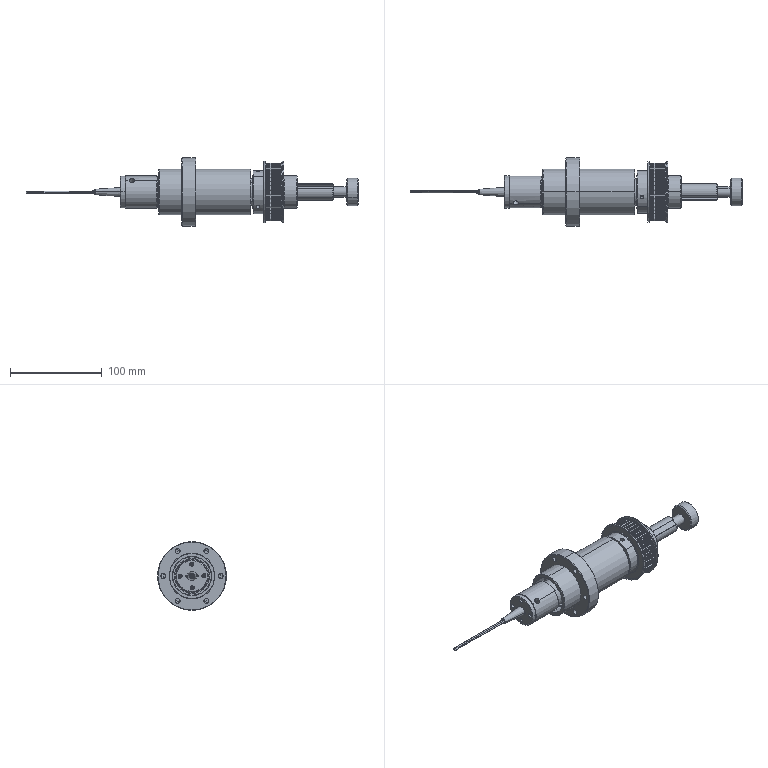Assembly | SolidWorks | mm | 15 component files | 15 solids | 1172 faces | box 362 x 75 x 75 mm | volume 344759 mm3 | cylinder 608 | torus 202 | cone 131 | plane 125 | sphere 104 | spline 2 | commonest cylinder face diameters 1.1 x98 0.5 x92 6.55 x86 59.16 x41 62.7 x40 5.5 x20 6 x20 3.4 x18
Bill of materials:
deep groove ball bearings gb | 4 |  | Ring-and-ball assembly geometry: an outer ring and an inner ring, concentric, with a row of spherical balls between them. The overall shape looks like a rolling-element ball bearing.
FlatKey6-175 | 1 | Alternative Material | Long, slender bar with a rectangular cross-section and five evenly spaced small round holes in a line along its length.
HTPA40S5M150_B_H30 | 1 | 45# | Toothed pulley-like rotational part: a cylindrical body with straight axial teeth around its outside, a thin flange at each end of the toothed section, and a smaller cylindrical hub on one side. It has a through bore with one keyway, and radial holes go through the hub wall.
JJDJR-3060-E-001 | 1 | 45# | Hollow cylindrical sleeve with a single circular flange placed off-center along its length. The flange has six through holes on a bolt circle.
JJDJR-3060-E-002 | 1 | 40Cr | Long hollow tube with a larger-diameter collar at one end, a row of small radial holes along its length, a slot near the other end, and a keyed bore.
JJDJR-3060-E-003 | 1 | 45# | Thick annular ring with chamfered outer edges, a central bore, and eight axial through holes evenly spaced around it.
JJDJR-3060-E-004 | 1 | 40Cr | Long shaft with a flat along its body, a smaller-diameter pin at one end with an axial hole, and a notched end block with small cross holes at the other end.
JJDJR-3060-E-005 | 1 | Tungsten Alloy | Thick plain washer- or spacer-like ring with chamfered outer edges and a small central through hole.
JJDJR-3060-E-006 | 1 | 40Cr | Small block with one convex curved face and a stepped rectangular tongue on the opposite side, pierced by two counterbored holes.
JJDJR-3060-E-007 | 1 | 40Cr | Circular flange with a long tapered conical shank on one side and a short stepped pilot boss on the other side.
JJDJR-3060-E-025 | 1 | Aluminum Alloy | Long thin rod with a slightly larger cylindrical hub at one end. The hub has a flat or notch, and the opposite end has a chamfered, slightly tapered tip.
Key6X6-36 | 1 | Alternative Material | Small rectangular bar with fully rounded ends (obround outline) and small chamfers along the edges.
Mates:
1. coincident | JJDJR-3060-E-001-1 face at (-89.59, -8.263, -16.52) dir (-1, 0, 0) | deep groove ball bearings gb-1 face at (-89.59, -41.121, -21.847) dir (1, 0, 0)
2. concentric | JJDJR-3060-E-001-1 face at (-103.59, -29.263, -16.52) dir (-1, 0, 0) r 21 | deep groove ball bearings gb-1 face at (-102.301, -29.263, -16.52) dir (-1, 0, 0) r 13
3. concentric | JJDJR-3060-E-001-1 face at (-103.59, -29.263, -16.52) dir (-1, 0, 0) r 21 | deep groove ball bearings gb-2 face at (-110.301, -29.263, -16.52) dir (-1, 0, 0) r 13
4. coincident | JJDJR-3060-E-001-1 face at (-17.59, -8.263, -16.52) dir (1, 0, 0) | deep groove ball bearings gb-3 face at (-17.59, -16.263, -16.52) dir (-1, 0, 0)
5. concentric | JJDJR-3060-E-001-1 face at (-103.59, -29.263, -16.52) dir (-1, 0, 0) r 21 | deep groove ball bearings gb-3 face at (-22.301, -29.263, -16.52) dir (-1, 0, 0) r 13
6. coincident | JJDJR-3060-E-002-1 face at (22.41, -37.957, -24.791) dir (0, -0.7245, -0.6892) | Key6X6-36-1 face at (22.41, -37.957, -24.791) dir (0, 0.7245, 0.6892)
7. concentric | JJDJR-3060-E-002-1 face at (34.41, -29.562, -28.516) dir (1, 0, 0) r 1.25 | JJDJR-3060-E-003-1 face at (47.41, -29.562, -28.516) dir (1, 0, 0) r 1.7
8. concentric | JJDJR-3060-E-002-1 face at (-140.59, -28.938, -3.524) dir (-1, 0, 0) r 1.65 | JJDJR-3060-E-007-1 face at (-137.59, -28.938, -3.524) dir (-1, 0, 0) r 2.25
9. concentric | JJDJR-3060-E-002-1 face at (22.41, -45.202, -31.684) dir (0, 0.7245, 0.6892) r 3 | Key6X6-36-1 face at (22.41, -42.304, -28.927) dir (0, 0.7245, 0.6892) r 3
10. concentric | JJDJR-3060-E-002-1 face at (-1.59, -45.202, -31.684) dir (0, 0.7245, 0.6892) r 3 | Key6X6-36-1 face at (-1.59, -42.304, -28.927) dir (0, 0.7245, 0.6892) r 3
11. concentric | JJDJR-3060-E-002-1 face at (-140.59, -29.263, -16.52) dir (-1, 0, 0) r 15 | deep groove ball bearings gb-2 face at (-108.562, -29.263, -16.52) dir (-1, 0, 0) r 5
12. concentric | JJDJR-3060-E-002-1 face at (-140.59, -29.263, -16.52) dir (-1, 0, 0) r 15 | HTPA40S5M150_B_H30-2 face at (-1.59, -29.263, -16.52) dir (1, 0, 0) r 15
13. coincident | JJDJR-3060-E-002-1 face at (-140.59, -33.61, -20.656) dir (-1, 0, 0) | JJDJR-3060-E-007-1 face at (-140.59, -29.038, -7.523) dir (1, 0, 0)
14. concentric | JJDJR-3060-E-002-1 face at (-140.59, -29.587, -29.516) dir (-1, 0, 0) r 1.65 | JJDJR-3060-E-007-1 face at (-137.59, -29.587, -29.516) dir (-1, 0, 0) r 2.25
15. coincident | JJDJR-3060-E-002-1 face at (-105.59, -41.942, -28.582) dir (1, 0, 0) | deep groove ball bearings gb-2 face at (-105.59, -36.929, -16.52) dir (-1, 0, 0)
16. concentric | JJDJR-3060-E-002-1 face at (34.41, -28.963, -4.524) dir (1, 0, 0) r 1.25 | JJDJR-3060-E-003-1 face at (47.41, -28.963, -4.524) dir (1, 0, 0) r 1.7
17. coincident | JJDJR-3060-E-004-1 face at (101.41, -29.263, -16.52) dir (1, 0, 0) | JJDJR-3060-E-005-1 face at (101.41, -29.263, -16.52) dir (-1, 0, 0)
18. coincident | JJDJR-3060-E-004-1 face at (101.41, -29.263, -16.52) dir (1, 0, 0) | JJDJR-3060-E-005-1 face at (101.41, -29.263, -16.52) dir (-1, 0, 0)
19. concentric | JJDJR-3060-E-004-1 face at (101.41, -29.263, -16.52) dir (1, 0, 0) r 2.5 | JJDJR-3060-E-005-1 face at (113.41, -29.263, -16.52) dir (1, 0, 0) r 3.3
20. concentric | JJDJR-3060-E-004-1 face at (-138.59, -29.263, -16.52) dir (-1, 0, 0) r 3 | JJDJR-3060-E-025-1 face at (-62.847, -29.263, -16.52) dir (1, 0, 0) r 3
21. coincident | JJDJR-3060-E-004-1 face at (-128.59, -36.508, -23.413) dir (0, -0.6892, 0.7245) | JJDJR-3060-E-006-1 face at (-118.59, -27.071, -14.435) dir (0, 0.6892, -0.7245)
22. concentric | JJDJR-3060-E-004-1 face at (-123.59, -25.64, -13.074) dir (0, -0.6892, 0.7245) r 1.025 | JJDJR-3060-E-006-1 face at (-123.59, -31.843, -6.553) dir (0, -0.6892, 0.7245) r 1.4
23. concentric | JJDJR-3060-E-004-1 face at (-123.59, -32.885, -19.966) dir (0, -0.6892, 0.7245) r 1.025 | JJDJR-3060-E-006-1 face at (-123.59, -39.089, -13.446) dir (0, -0.6892, 0.7245) r 1.4
24. coincident | JJDJR-3060-E-004-1 face at (-128.59, -36.508, -23.413) dir (1, 0, 0) | JJDJR-3060-E-025-1 face at (-128.59, -26.674, -11.987) dir (1, 0, 0)
25. distance | JJDJR-3060-E-025-1 face at (-248.59, -31.331, -14.347) dir (-1, 0, 0) | JJDJR-3060-E-007-1 face at (-173.59, -29.225, -15.021) dir (-1, 0, 0)
26. coincident | JJDJR-3060-E-003-1 face at (32.41, -38.31, -16.294) dir (-1, 0, 0) | HTPA40S5M150_B_H30-2 face at (32.41, -47.231, -33.613) dir (1, 0, 0)
27. coincident | Key6X6-36-1 face at (22.41, -40.237, -31.1) dir (0, 0.6892, -0.7245) | HTPA40S5M150_B_H30-2 face at (32.41, -34.159, -25.319) dir (0, -0.6892, 0.7245)
28. coincident | deep groove ball bearings gb-1 face at (-97.59, -41.121, -21.847) dir (-1, 0, 0) | deep groove ball bearings gb-2 face at (-97.59, -42.263, -16.52) dir (1, 0, 0)
29. coincident | deep groove ball bearings gb-3 face at (-9.59, -16.263, -16.52) dir (1, 0, 0) | deep groove ball bearings gb-4 face at (-9.59, -16.263, -16.52) dir (-1, 0, 0)
30. concentric | deep groove ball bearings gb-3 face at (-22.301, -29.263, -16.52) dir (-1, 0, 0) r 13 | deep groove ball bearings gb-4 face at (-14.301, -29.263, -16.52) dir (-1, 0, 0) r 13
31. coincident | deep groove ball bearings gb-4 face at (-1.59, -24.263, -16.52) dir (1, 0, 0) | HTPA40S5M150_B_H30-2 face at (-1.59, -40.276, -26.997) dir (-1, 0, 0)
32. concentric | JJDJR-3060-E-002-1 face at (34.41, -29.263, -16.52) dir (-1, 0, 0) r 9 | JJDJR-3060-E-004-1 face at (101.41, -29.263, -16.52) dir (1, 0, 0) r 9
33. parallel | JJDJR-3060-E-004-1 face at (-128.59, -36.508, -23.413) dir (0, -0.6892, 0.7245) | JJDJR-3060-E-025-1 face at (-118.59, -26.674, -11.987) dir (0, -0.6892, 0.7245)
34. coincident | JJDJR-3060-E-002-1 face at (-140.59, -33.982, -7.207) dir (0, 0.6892, -0.7245) | FlatKey6-175-1 face at (34.41, -38.329, -11.343) dir (0, -0.6892, 0.7245)
35. concentric | JJDJR-3060-E-002-1 face at (-133.09, -41.325, -3.841) dir (0, -0.6892, 0.7245) r 1.7 | FlatKey6-175-1 face at (-133.09, -33.192, -12.39) dir (0, 0.6892, -0.7245) r 1.25
36. width | JJDJR-3060-E-004-1 face at (-138.59, -34.853, -6.291) dir (0, -0.7245, -0.6892) | JJDJR-3060-E-004-1 face at (-138.59, -39.2, -10.427) dir (0, 0.7245, 0.6892) | FlatKey6-175-1 face at (-140.59, -31.018, -10.323) dir (0, 0.7245, 0.6892) | FlatKey6-175-1 face at (-140.59, -35.365, -14.458) dir (0, -0.7245, -0.6892)